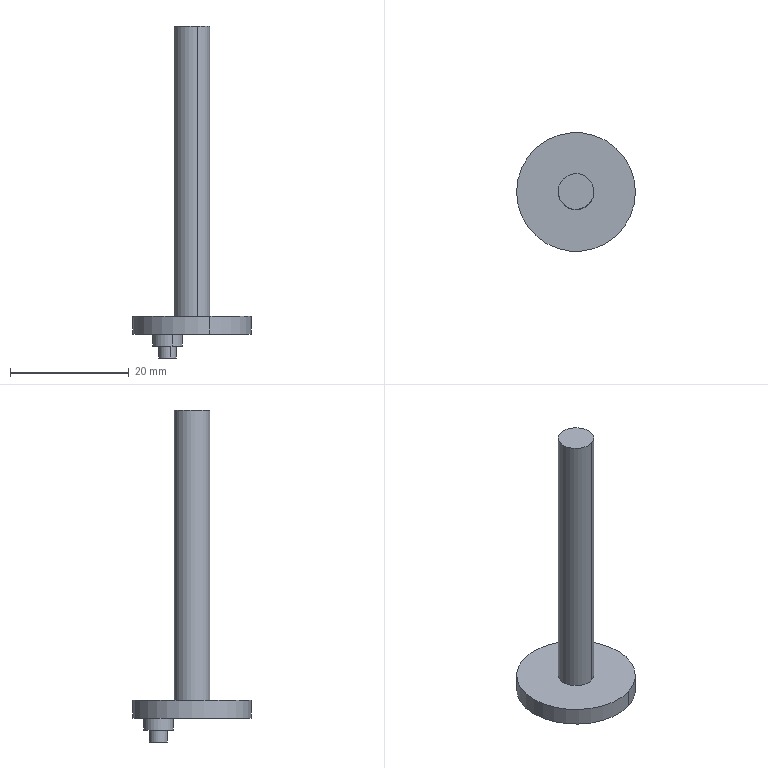Component | SolidWorks | 5-1 | 1 solid | 13 faces | box 20 x 20 x 55.88 mm | volume 2378 mm3 | cylinder 8 | plane 5 | commonest cylinder face diameters 3 x2 5 x2 20 x2 6 x2
build123d program:
from build123d import *

# Parameters (mm, degrees)
SKETCH1_R           = 10
BOSS_EXTRUDE1_DEPTH = 3
SKETCH2_R           = 2.5
BOSS_EXTRUDE2_DEPTH = 2
SKETCH3_R           = 1.5
BOSS_EXTRUDE3_DEPTH = 2
SKETCH4_R           = 3
BOSS_EXTRUDE4_DEPTH = 50
CUT_EXTRUDE1_START  = -2.12
SKETCH5_R           = 3
CUT_EXTRUDE1_DEPTH  = 2.12
SKETCH6_R           = 3
BOSS_EXTRUDE5_DEPTH = 1


with BuildPart() as part:
    # Sketch1 → Boss-Extrude1 (new body)
    with BuildSketch(Plane.XY):
        with Locations((9.395, 17.038)):
            Circle(SKETCH1_R)
    extrude(amount=BOSS_EXTRUDE1_DEPTH)

    # Sketch2 → Boss-Extrude2 (add)
    with BuildSketch(Plane.XY.offset(3)):
        with Locations((16.034, 14.819)):
            Circle(SKETCH2_R)
    extrude(amount=BOSS_EXTRUDE2_DEPTH)

    # Sketch3 → Boss-Extrude3 (add)
    with BuildSketch(Plane.XY.offset(5)):
        with Locations((16.034, 14.819)):
            Circle(SKETCH3_R)
    extrude(amount=BOSS_EXTRUDE3_DEPTH)

    # Sketch4 → Boss-Extrude4 (add)
    with BuildSketch(Plane(origin=(0, 0, 0), x_dir=(-1, 0, 0), z_dir=(0, 0, -1))):
        with Locations(Location((-9.395, 17.038, 0), (0, 0, 180))):
            Circle(SKETCH4_R)
    extrude(amount=BOSS_EXTRUDE4_DEPTH)

    # Sketch5 → Cut-Extrude1 (cut)
    with BuildSketch(Plane(origin=(0, 0, -50), x_dir=(-1, 0, 0), z_dir=(0, 0, -1)).offset(CUT_EXTRUDE1_START)):
        with Locations(Location((-9.395, 17.038, 0), (0, 0, 180))):
            Circle(SKETCH5_R)
    extrude(amount=CUT_EXTRUDE1_DEPTH, mode=Mode.SUBTRACT)

    # Sketch6 → Boss-Extrude5 (add)
    with BuildSketch(Plane(origin=(0, 0, -47.88), x_dir=(-1, 0, 0), z_dir=(0, 0, -1))):
        with Locations(Location((-9.395, 17.038, 0), (0, 0, 180))):
            Circle(SKETCH6_R)
    extrude(amount=BOSS_EXTRUDE5_DEPTH)


solid = part.part

# Placed as in the assembly
solid = solid.moved(Location((55.928, -7.071, -22.938), (180, 0, -107.592)))
STEP:
#1=COLOUR_RGB('',0.7922,0.8196,0.9333);
#2=FILL_AREA_STYLE_COLOUR('',#1);
#3=FILL_AREA_STYLE('',(#2));
#4=SURFACE_STYLE_FILL_AREA(#3);
#5=SURFACE_SIDE_STYLE('',(#4));
#6=SURFACE_STYLE_USAGE(.BOTH.,#5);
#7=PRESENTATION_STYLE_ASSIGNMENT((#6));
#8=CARTESIAN_POINT('',(2.549,0.556,-1.179));
#9=VERTEX_POINT('',#8);
#10=CARTESIAN_POINT('',(2.585,0.4434,-1.179));
#11=VERTEX_POINT('',#10);
#12=CARTESIAN_POINT('',(2.567,0.4997,-1.179));
#13=DIRECTION('',(0.,-0.,-1.));
#14=DIRECTION('',(-0.3022,0.9532,0.));
#15=AXIS2_PLACEMENT_3D('',#12,#13,#14);
#16=CIRCLE('',#15,0.05906);
#17=EDGE_CURVE('',#9,#11,#16,.T.);
#18=ORIENTED_EDGE('',*,*,#17,.F.);
#19=CARTESIAN_POINT('',(2.549,0.556,-1.1));
#20=VERTEX_POINT('',#19);
#21=CARTESIAN_POINT('',(2.549,0.556,-1.179));
#22=DIRECTION('',(-0.,0.,1.));
#23=VECTOR('',#22,39.37);
#24=LINE('',#21,#23);
#25=EDGE_CURVE('',#9,#20,#24,.T.);
#26=ORIENTED_EDGE('',*,*,#25,.T.);
#27=CARTESIAN_POINT('',(2.585,0.4434,-1.1));
#28=VERTEX_POINT('',#27);
#29=CARTESIAN_POINT('',(2.567,0.4997,-1.1));
#30=DIRECTION('',(0.,-0.,-1.));
#31=DIRECTION('',(-0.3022,0.9532,0.));
#32=AXIS2_PLACEMENT_3D('',#29,#30,#31);
#33=CIRCLE('',#32,0.05906);
#34=EDGE_CURVE('',#20,#28,#33,.T.);
#35=ORIENTED_EDGE('',*,*,#34,.T.);
#36=CARTESIAN_POINT('',(2.585,0.4434,-1.179));
#37=DIRECTION('',(-0.,0.,1.));
#38=VECTOR('',#37,39.37);
#39=LINE('',#36,#38);
#40=EDGE_CURVE('',#11,#28,#39,.T.);
#41=ORIENTED_EDGE('',*,*,#40,.F.);
#42=EDGE_LOOP('',(#18,#26,#35,#41));
#43=FACE_OUTER_BOUND('',#42,.T.);
#44=CARTESIAN_POINT('',(2.567,0.4997,-1.179));
#45=DIRECTION('',(-0.,0.,1.));
#46=DIRECTION('',(0.3022,-0.9532,0.));
#47=AXIS2_PLACEMENT_3D('',#44,#45,#46);
#48=CYLINDRICAL_SURFACE('',#47,0.05906);
#49=ADVANCED_FACE('',(#43),#48,.T.);
#50=CARTESIAN_POINT('',(2.537,0.5935,-1.1));
#51=VERTEX_POINT('',#50);
#52=CARTESIAN_POINT('',(2.597,0.4059,-1.1));
#53=VERTEX_POINT('',#52);
#54=CARTESIAN_POINT('',(2.567,0.4997,-1.1));
#55=DIRECTION('',(0.,-0.,-1.));
#56=DIRECTION('',(-0.3022,0.9532,0.));
#57=AXIS2_PLACEMENT_3D('',#54,#55,#56);
#58=CIRCLE('',#57,0.09843);
#59=EDGE_CURVE('',#51,#53,#58,.T.);
#60=ORIENTED_EDGE('',*,*,#59,.F.);
#61=CARTESIAN_POINT('',(2.537,0.5935,-1.021));
#62=VERTEX_POINT('',#61);
#63=CARTESIAN_POINT('',(2.537,0.5935,-1.1));
#64=DIRECTION('',(-0.,0.,1.));
#65=VECTOR('',#64,39.37);
#66=LINE('',#63,#65);
#67=EDGE_CURVE('',#51,#62,#66,.T.);
#68=ORIENTED_EDGE('',*,*,#67,.T.);
#69=CARTESIAN_POINT('',(2.597,0.4059,-1.021));
#70=VERTEX_POINT('',#69);
#71=CARTESIAN_POINT('',(2.567,0.4997,-1.021));
#72=DIRECTION('',(0.,-0.,-1.));
#73=DIRECTION('',(-0.3022,0.9532,0.));
#74=AXIS2_PLACEMENT_3D('',#71,#72,#73);
#75=CIRCLE('',#74,0.09843);
#76=EDGE_CURVE('',#62,#70,#75,.T.);
#77=ORIENTED_EDGE('',*,*,#76,.T.);
#78=CARTESIAN_POINT('',(2.597,0.4059,-1.1));
#79=DIRECTION('',(-0.,0.,1.));
#80=VECTOR('',#79,39.37);
#81=LINE('',#78,#80);
#82=EDGE_CURVE('',#53,#70,#81,.T.);
#83=ORIENTED_EDGE('',*,*,#82,.F.);
#84=EDGE_LOOP('',(#60,#68,#77,#83));
#85=FACE_OUTER_BOUND('',#84,.T.);
#86=CARTESIAN_POINT('',(2.567,0.4997,-1.1));
#87=DIRECTION('',(-0.,0.,1.));
#88=DIRECTION('',(0.3022,-0.9532,0.));
#89=AXIS2_PLACEMENT_3D('',#86,#87,#88);
#90=CYLINDRICAL_SURFACE('',#89,0.09843);
#91=ADVANCED_FACE('',(#85),#90,.T.);
#92=CARTESIAN_POINT('',(2.611,0.6522,-1.021));
#93=VERTEX_POINT('',#92);
#94=CARTESIAN_POINT('',(2.848,-0.09836,-1.021));
#95=VERTEX_POINT('',#94);
#96=CARTESIAN_POINT('',(2.73,0.2769,-1.021));
#97=DIRECTION('',(0.,-0.,-1.));
#98=DIRECTION('',(-0.3022,0.9532,0.));
#99=AXIS2_PLACEMENT_3D('',#96,#97,#98);
#100=CIRCLE('',#99,0.3937);
#101=EDGE_CURVE('',#93,#95,#100,.T.);
#102=ORIENTED_EDGE('',*,*,#101,.F.);
#103=CARTESIAN_POINT('',(2.611,0.6522,-0.9031));
#104=VERTEX_POINT('',#103);
#105=CARTESIAN_POINT('',(2.611,0.6522,-1.021));
#106=DIRECTION('',(-0.,0.,1.));
#107=VECTOR('',#106,39.37);
#108=LINE('',#105,#107);
#109=EDGE_CURVE('',#93,#104,#108,.T.);
#110=ORIENTED_EDGE('',*,*,#109,.T.);
#111=CARTESIAN_POINT('',(2.848,-0.09836,-0.9031));
#112=VERTEX_POINT('',#111);
#113=CARTESIAN_POINT('',(2.73,0.2769,-0.9031));
#114=DIRECTION('',(0.,-0.,-1.));
#115=DIRECTION('',(-0.3022,0.9532,0.));
#116=AXIS2_PLACEMENT_3D('',#113,#114,#115);
#117=CIRCLE('',#116,0.3937);
#118=EDGE_CURVE('',#104,#112,#117,.T.);
#119=ORIENTED_EDGE('',*,*,#118,.T.);
#120=CARTESIAN_POINT('',(2.848,-0.09836,-1.021));
#121=DIRECTION('',(-0.,0.,1.));
#122=VECTOR('',#121,39.37);
#123=LINE('',#120,#122);
#124=EDGE_CURVE('',#95,#112,#123,.T.);
#125=ORIENTED_EDGE('',*,*,#124,.F.);
#126=EDGE_LOOP('',(#102,#110,#119,#125));
#127=FACE_OUTER_BOUND('',#126,.T.);
#128=CARTESIAN_POINT('',(2.73,0.2769,-1.021));
#129=DIRECTION('',(-0.,0.,1.));
#130=DIRECTION('',(0.3022,-0.9532,0.));
#131=AXIS2_PLACEMENT_3D('',#128,#129,#130);
#132=CYLINDRICAL_SURFACE('',#131,0.3937);
#133=ADVANCED_FACE('',(#127),#132,.T.);
#134=CARTESIAN_POINT('',(2.765,0.1643,1.021));
#135=VERTEX_POINT('',#134);
#136=CARTESIAN_POINT('',(2.694,0.3895,1.021));
#137=VERTEX_POINT('',#136);
#138=CARTESIAN_POINT('',(2.73,0.2769,1.021));
#139=DIRECTION('',(-0.,0.,1.));
#140=DIRECTION('',(0.3022,-0.9532,0.));
#141=AXIS2_PLACEMENT_3D('',#138,#139,#140);
#142=CIRCLE('',#141,0.1181);
#143=EDGE_CURVE('',#135,#137,#142,.T.);
#144=ORIENTED_EDGE('',*,*,#143,.F.);
#145=CARTESIAN_POINT('',(2.765,0.1643,-0.9031));
#146=VERTEX_POINT('',#145);
#147=CARTESIAN_POINT('',(2.765,0.1643,1.065));
#148=DIRECTION('',(0.,-0.,-1.));
#149=VECTOR('',#148,39.37);
#150=LINE('',#147,#149);
#151=EDGE_CURVE('',#135,#146,#150,.T.);
#152=ORIENTED_EDGE('',*,*,#151,.T.);
#153=CARTESIAN_POINT('',(2.694,0.3895,-0.9031));
#154=VERTEX_POINT('',#153);
#155=CARTESIAN_POINT('',(2.73,0.2769,-0.9031));
#156=DIRECTION('',(-0.,0.,1.));
#157=DIRECTION('',(-0.3022,0.9532,0.));
#158=AXIS2_PLACEMENT_3D('',#155,#156,#157);
#159=CIRCLE('',#158,0.1181);
#160=EDGE_CURVE('',#146,#154,#159,.T.);
#161=ORIENTED_EDGE('',*,*,#160,.T.);
#162=CARTESIAN_POINT('',(2.694,0.3895,1.065));
#163=DIRECTION('',(0.,-0.,-1.));
#164=VECTOR('',#163,39.37);
#165=LINE('',#162,#164);
#166=EDGE_CURVE('',#137,#154,#165,.T.);
#167=ORIENTED_EDGE('',*,*,#166,.F.);
#168=EDGE_LOOP('',(#144,#152,#161,#167));
#169=FACE_OUTER_BOUND('',#168,.T.);
#170=CARTESIAN_POINT('',(2.73,0.2769,1.065));
#171=DIRECTION('',(0.,-0.,-1.));
#172=DIRECTION('',(-0.3022,0.9532,0.));
#173=AXIS2_PLACEMENT_3D('',#170,#171,#172);
#174=CYLINDRICAL_SURFACE('',#173,0.1181);
#175=ADVANCED_FACE('',(#169),#174,.T.);
#176=ORIENTED_EDGE('',*,*,#151,.F.);
#177=CARTESIAN_POINT('',(2.73,0.2769,1.021));
#178=DIRECTION('',(-0.,0.,1.));
#179=DIRECTION('',(0.3022,-0.9532,0.));
#180=AXIS2_PLACEMENT_3D('',#177,#178,#179);
#181=CIRCLE('',#180,0.1181);
#182=EDGE_CURVE('',#137,#135,#181,.T.);
#183=ORIENTED_EDGE('',*,*,#182,.F.);
#184=ORIENTED_EDGE('',*,*,#166,.T.);
#185=CARTESIAN_POINT('',(2.73,0.2769,-0.9031));
#186=DIRECTION('',(-0.,0.,1.));
#187=DIRECTION('',(-0.3022,0.9532,0.));
#188=AXIS2_PLACEMENT_3D('',#185,#186,#187);
#189=CIRCLE('',#188,0.1181);
#190=EDGE_CURVE('',#154,#146,#189,.T.);
#191=ORIENTED_EDGE('',*,*,#190,.T.);
#192=EDGE_LOOP('',(#176,#183,#184,#191));
#193=FACE_OUTER_BOUND('',#192,.T.);
#194=CARTESIAN_POINT('',(2.73,0.2769,1.065));
#195=DIRECTION('',(0.,-0.,-1.));
#196=DIRECTION('',(-0.3022,0.9532,0.));
#197=AXIS2_PLACEMENT_3D('',#194,#195,#196);
#198=CYLINDRICAL_SURFACE('',#197,0.1181);
#199=ADVANCED_FACE('',(#193),#198,.T.);
#200=CARTESIAN_POINT('',(2.73,0.2769,-0.9031));
#201=DIRECTION('',(0.,-0.,-1.));
#202=DIRECTION('',(-0.3022,0.9532,0.));
#203=AXIS2_PLACEMENT_3D('',#200,#201,#202);
#204=CIRCLE('',#203,0.3937);
#205=EDGE_CURVE('',#112,#104,#204,.T.);
#206=ORIENTED_EDGE('',*,*,#205,.F.);
#207=ORIENTED_EDGE('',*,*,#118,.F.);
#208=EDGE_LOOP('',(#206,#207));
#209=FACE_OUTER_BOUND('',#208,.T.);
#210=ORIENTED_EDGE('',*,*,#190,.F.);
#211=ORIENTED_EDGE('',*,*,#160,.F.);
#212=EDGE_LOOP('',(#210,#211));
#213=FACE_BOUND('',#212,.T.);
#214=CARTESIAN_POINT('',(2.73,0.2769,-0.9031));
#215=DIRECTION('',(0.,-0.,-1.));
#216=DIRECTION('',(-0.3022,0.9532,-0.));
#217=AXIS2_PLACEMENT_3D('',#214,#215,#216);
#218=PLANE('',#217);
#219=ADVANCED_FACE('',(#209,#213),#218,.F.);
#220=CARTESIAN_POINT('',(2.567,0.4997,-1.1));
#221=DIRECTION('',(0.,-0.,-1.));
#222=DIRECTION('',(-0.3022,0.9532,0.));
#223=AXIS2_PLACEMENT_3D('',#220,#221,#222);
#224=CIRCLE('',#223,0.09843);
#225=EDGE_CURVE('',#53,#51,#224,.T.);
#226=ORIENTED_EDGE('',*,*,#225,.T.);
#227=ORIENTED_EDGE('',*,*,#59,.T.);
#228=EDGE_LOOP('',(#226,#227));
#229=FACE_OUTER_BOUND('',#228,.T.);
#230=CARTESIAN_POINT('',(2.567,0.4997,-1.1));
#231=DIRECTION('',(0.,-0.,-1.));
#232=DIRECTION('',(-0.3022,0.9532,0.));
#233=AXIS2_PLACEMENT_3D('',#230,#231,#232);
#234=CIRCLE('',#233,0.05906);
#235=EDGE_CURVE('',#28,#20,#234,.T.);
#236=ORIENTED_EDGE('',*,*,#235,.F.);
#237=ORIENTED_EDGE('',*,*,#34,.F.);
#238=EDGE_LOOP('',(#236,#237));
#239=FACE_BOUND('',#238,.T.);
#240=CARTESIAN_POINT('',(2.567,0.4997,-1.1));
#241=DIRECTION('',(0.,-0.,-1.));
#242=DIRECTION('',(-0.3022,0.9532,-0.));
#243=AXIS2_PLACEMENT_3D('',#240,#241,#242);
#244=PLANE('',#243);
#245=ADVANCED_FACE('',(#229,#239),#244,.T.);
#246=CARTESIAN_POINT('',(2.73,0.2769,-1.021));
#247=DIRECTION('',(0.,-0.,-1.));
#248=DIRECTION('',(-0.3022,0.9532,0.));
#249=AXIS2_PLACEMENT_3D('',#246,#247,#248);
#250=CIRCLE('',#249,0.3937);
#251=EDGE_CURVE('',#95,#93,#250,.T.);
#252=ORIENTED_EDGE('',*,*,#251,.T.);
#253=ORIENTED_EDGE('',*,*,#101,.T.);
#254=EDGE_LOOP('',(#252,#253));
#255=FACE_OUTER_BOUND('',#254,.T.);
#256=CARTESIAN_POINT('',(2.567,0.4997,-1.021));
#257=DIRECTION('',(0.,-0.,-1.));
#258=DIRECTION('',(-0.3022,0.9532,0.));
#259=AXIS2_PLACEMENT_3D('',#256,#257,#258);
#260=CIRCLE('',#259,0.09843);
#261=EDGE_CURVE('',#70,#62,#260,.T.);
#262=ORIENTED_EDGE('',*,*,#261,.F.);
#263=ORIENTED_EDGE('',*,*,#76,.F.);
#264=EDGE_LOOP('',(#262,#263));
#265=FACE_BOUND('',#264,.T.);
#266=CARTESIAN_POINT('',(2.73,0.2769,-1.021));
#267=DIRECTION('',(0.,-0.,-1.));
#268=DIRECTION('',(-0.3022,0.9532,-0.));
#269=AXIS2_PLACEMENT_3D('',#266,#267,#268);
#270=PLANE('',#269);
#271=ADVANCED_FACE('',(#255,#265),#270,.T.);
#272=ORIENTED_EDGE('',*,*,#109,.F.);
#273=ORIENTED_EDGE('',*,*,#251,.F.);
#274=ORIENTED_EDGE('',*,*,#124,.T.);
#275=ORIENTED_EDGE('',*,*,#205,.T.);
#276=EDGE_LOOP('',(#272,#273,#274,#275));
#277=FACE_OUTER_BOUND('',#276,.T.);
#278=CARTESIAN_POINT('',(2.73,0.2769,-1.021));
#279=DIRECTION('',(-0.,0.,1.));
#280=DIRECTION('',(0.3022,-0.9532,0.));
#281=AXIS2_PLACEMENT_3D('',#278,#279,#280);
#282=CYLINDRICAL_SURFACE('',#281,0.3937);
#283=ADVANCED_FACE('',(#277),#282,.T.);
#284=ORIENTED_EDGE('',*,*,#67,.F.);
#285=ORIENTED_EDGE('',*,*,#225,.F.);
#286=ORIENTED_EDGE('',*,*,#82,.T.);
#287=ORIENTED_EDGE('',*,*,#261,.T.);
#288=EDGE_LOOP('',(#284,#285,#286,#287));
#289=FACE_OUTER_BOUND('',#288,.T.);
#290=CARTESIAN_POINT('',(2.567,0.4997,-1.1));
#291=DIRECTION('',(-0.,0.,1.));
#292=DIRECTION('',(0.3022,-0.9532,0.));
#293=AXIS2_PLACEMENT_3D('',#290,#291,#292);
#294=CYLINDRICAL_SURFACE('',#293,0.09843);
#295=ADVANCED_FACE('',(#289),#294,.T.);
#296=ORIENTED_EDGE('',*,*,#25,.F.);
#297=CARTESIAN_POINT('',(2.567,0.4997,-1.179));
#298=DIRECTION('',(0.,-0.,-1.));
#299=DIRECTION('',(-0.3022,0.9532,0.));
#300=AXIS2_PLACEMENT_3D('',#297,#298,#299);
#301=CIRCLE('',#300,0.05906);
#302=EDGE_CURVE('',#11,#9,#301,.T.);
#303=ORIENTED_EDGE('',*,*,#302,.F.);
#304=ORIENTED_EDGE('',*,*,#40,.T.);
#305=ORIENTED_EDGE('',*,*,#235,.T.);
#306=EDGE_LOOP('',(#296,#303,#304,#305));
#307=FACE_OUTER_BOUND('',#306,.T.);
#308=CARTESIAN_POINT('',(2.567,0.4997,-1.179));
#309=DIRECTION('',(-0.,0.,1.));
#310=DIRECTION('',(0.3022,-0.9532,0.));
#311=AXIS2_PLACEMENT_3D('',#308,#309,#310);
#312=CYLINDRICAL_SURFACE('',#311,0.05906);
#313=ADVANCED_FACE('',(#307),#312,.T.);
#314=ORIENTED_EDGE('',*,*,#302,.T.);
#315=ORIENTED_EDGE('',*,*,#17,.T.);
#316=EDGE_LOOP('',(#314,#315));
#317=FACE_OUTER_BOUND('',#316,.T.);
#318=CARTESIAN_POINT('',(2.567,0.4997,-1.179));
#319=DIRECTION('',(0.,-0.,-1.));
#320=DIRECTION('',(-0.3022,0.9532,-0.));
#321=AXIS2_PLACEMENT_3D('',#318,#319,#320);
#322=PLANE('',#321);
#323=ADVANCED_FACE('',(#317),#322,.T.);
#324=ORIENTED_EDGE('',*,*,#182,.T.);
#325=ORIENTED_EDGE('',*,*,#143,.T.);
#326=EDGE_LOOP('',(#324,#325));
#327=FACE_OUTER_BOUND('',#326,.T.);
#328=CARTESIAN_POINT('',(2.73,0.2769,1.021));
#329=DIRECTION('',(-0.,0.,1.));
#330=DIRECTION('',(0.3022,-0.9532,0.));
#331=AXIS2_PLACEMENT_3D('',#328,#329,#330);
#332=PLANE('',#331);
#333=ADVANCED_FACE('',(#327),#332,.T.);
#334=CLOSED_SHELL('',(#49,#91,#133,#175,#199,#219,#245,#271,#283,#295,#313,#323,#333));
#335=MANIFOLD_SOLID_BREP('',#334);
#336=STYLED_ITEM('',(#7),#335);
#337=(LENGTH_UNIT()NAMED_UNIT(*)SI_UNIT($,.METRE.));
#338=LENGTH_MEASURE_WITH_UNIT(LENGTH_MEASURE(0.0254),#337);
#339=DIMENSIONAL_EXPONENTS(1.,0.,0.,0.,0.,0.,0.);
#340=(CONVERSION_BASED_UNIT('',#338)LENGTH_UNIT()NAMED_UNIT(#339));
#341=UNCERTAINTY_MEASURE_WITH_UNIT(LENGTH_MEASURE(0.00001),#340,'','');
#342=(NAMED_UNIT(*)PLANE_ANGLE_UNIT()SI_UNIT($,.RADIAN.));
#343=(NAMED_UNIT(*)SI_UNIT($,.STERADIAN.)SOLID_ANGLE_UNIT());
#344=(GEOMETRIC_REPRESENTATION_CONTEXT(3)GLOBAL_UNCERTAINTY_ASSIGNED_CONTEXT((#341))GLOBAL_UNIT_ASSIGNED_CONTEXT((#340,#342,#343))REPRESENTATION_CONTEXT('',''));
#345=MECHANICAL_DESIGN_GEOMETRIC_PRESENTATION_REPRESENTATION('',(#336),#344);
#346=CARTESIAN_POINT('',(0.,0.,0.));
#347=DIRECTION('',(0.,0.,1.));
#348=DIRECTION('',(1.,0.,0.));
#349=AXIS2_PLACEMENT_3D('',#346,#347,#348);
#350=(LENGTH_UNIT()NAMED_UNIT(*)SI_UNIT($,.METRE.));
#351=LENGTH_MEASURE_WITH_UNIT(LENGTH_MEASURE(0.0254),#350);
#352=DIMENSIONAL_EXPONENTS(1.,0.,0.,0.,0.,0.,0.);
#353=(CONVERSION_BASED_UNIT('',#351)LENGTH_UNIT()NAMED_UNIT(#352));
#354=UNCERTAINTY_MEASURE_WITH_UNIT(LENGTH_MEASURE(0.00001),#353,'','');
#355=(NAMED_UNIT(*)PLANE_ANGLE_UNIT()SI_UNIT($,.RADIAN.));
#356=(NAMED_UNIT(*)SI_UNIT($,.STERADIAN.)SOLID_ANGLE_UNIT());
#357=(GEOMETRIC_REPRESENTATION_CONTEXT(3)GLOBAL_UNCERTAINTY_ASSIGNED_CONTEXT((#354))GLOBAL_UNIT_ASSIGNED_CONTEXT((#353,#355,#356))REPRESENTATION_CONTEXT('',''));
#358=ADVANCED_BREP_SHAPE_REPRESENTATION('',(#335,#349),#357);
#359=PRESENTATION_LAYER_ASSIGNMENT('','',(#336));